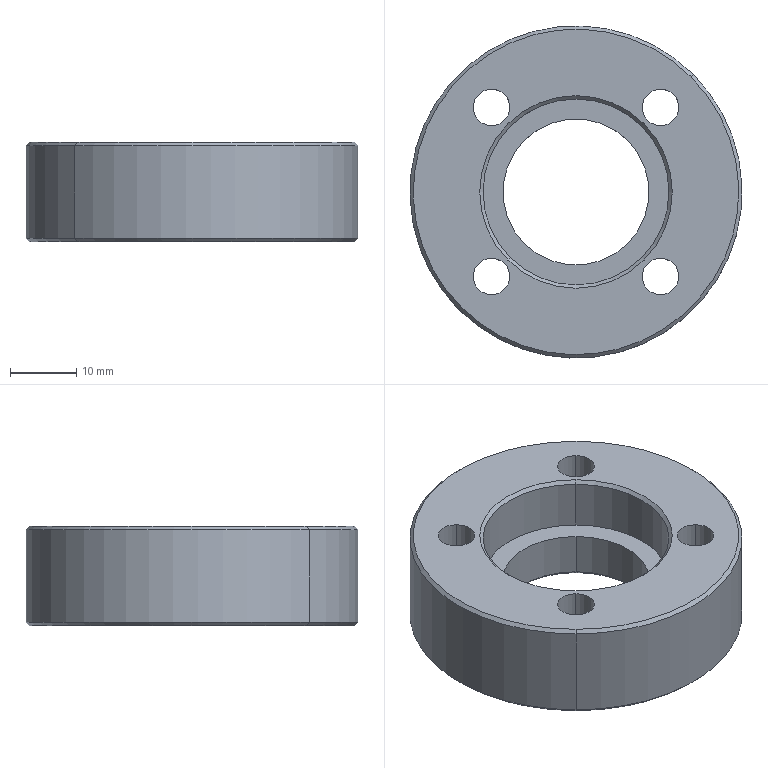Component | SolidWorks | SL010-LeftStreamline-1-1_SL010-2M-0112-000-2-1-1_SL010-LXFB-0102009-1-1 | 1 solid | 37 faces | box 50 x 50 x 15 mm | volume 19198 mm3 | cylinder 22 | cone 8 | plane 7 | commonest cylinder face diameters 10 x8 5.5 x8 22 x2 28 x2 50 x2 | material Aluminum-6061
STEP:
#1=COLOUR_RGB('',0.7922,0.8196,0.9333);
#2=FILL_AREA_STYLE_COLOUR('',#1);
#3=FILL_AREA_STYLE('',(#2));
#4=SURFACE_STYLE_FILL_AREA(#3);
#5=SURFACE_SIDE_STYLE('',(#4));
#6=SURFACE_STYLE_USAGE(.BOTH.,#5);
#7=PRESENTATION_STYLE_ASSIGNMENT((#6));
#8=CARTESIAN_POINT('',(-7.28,-6.882,-25.927));
#9=VERTEX_POINT('',#8);
#10=CARTESIAN_POINT('',(-6.5,-6.103,-25.927));
#11=VERTEX_POINT('',#10);
#12=CARTESIAN_POINT('',(-6.89,-6.492,-25.927));
#13=DIRECTION('',(0.,-0.,1.));
#14=DIRECTION('',(0.7071,0.7071,0.));
#15=AXIS2_PLACEMENT_3D('',#12,#13,#14);
#16=CIRCLE('',#15,0.5512);
#17=EDGE_CURVE('',#9,#11,#16,.T.);
#18=ORIENTED_EDGE('',*,*,#17,.F.);
#19=CARTESIAN_POINT('',(-7.293,-6.896,-25.907));
#20=VERTEX_POINT('',#19);
#21=CARTESIAN_POINT('',(-7.28,-6.882,-25.927));
#22=DIRECTION('',(-0.5,-0.5,0.7071));
#23=VECTOR('',#22,39.37);
#24=LINE('',#21,#23);
#25=EDGE_CURVE('',#9,#20,#24,.T.);
#26=ORIENTED_EDGE('',*,*,#25,.T.);
#27=CARTESIAN_POINT('',(-6.486,-6.089,-25.907));
#28=VERTEX_POINT('',#27);
#29=CARTESIAN_POINT('',(-6.89,-6.492,-25.907));
#30=DIRECTION('',(-0.,0.,-1.));
#31=DIRECTION('',(0.7071,0.7071,0.));
#32=AXIS2_PLACEMENT_3D('',#29,#30,#31);
#33=CIRCLE('',#32,0.5709);
#34=EDGE_CURVE('',#28,#20,#33,.T.);
#35=ORIENTED_EDGE('',*,*,#34,.F.);
#36=CARTESIAN_POINT('',(-6.5,-6.103,-25.927));
#37=DIRECTION('',(0.5,0.5,0.7071));
#38=VECTOR('',#37,39.37);
#39=LINE('',#36,#38);
#40=EDGE_CURVE('',#11,#28,#39,.T.);
#41=ORIENTED_EDGE('',*,*,#40,.F.);
#42=EDGE_LOOP('',(#18,#26,#35,#41));
#43=FACE_OUTER_BOUND('',#42,.T.);
#44=CARTESIAN_POINT('',(-6.89,-6.492,-25.927));
#45=DIRECTION('',(0.,-0.,1.));
#46=DIRECTION('',(0.7071,0.7071,0.));
#47=AXIS2_PLACEMENT_3D('',#44,#45,#46);
#48=CONICAL_SURFACE('',#47,0.5512,0.7854);
#49=ADVANCED_FACE('',(#43),#48,.F.);
#50=CARTESIAN_POINT('',(-6.584,-6.186,-26.478));
#51=VERTEX_POINT('',#50);
#52=CARTESIAN_POINT('',(-7.196,-6.799,-26.478));
#53=VERTEX_POINT('',#52);
#54=CARTESIAN_POINT('',(-6.89,-6.492,-26.478));
#55=DIRECTION('',(-0.,0.,-1.));
#56=DIRECTION('',(0.7071,0.7071,0.));
#57=AXIS2_PLACEMENT_3D('',#54,#55,#56);
#58=CIRCLE('',#57,0.4331);
#59=EDGE_CURVE('',#51,#53,#58,.T.);
#60=ORIENTED_EDGE('',*,*,#59,.F.);
#61=CARTESIAN_POINT('',(-6.57,-6.172,-26.497));
#62=VERTEX_POINT('',#61);
#63=CARTESIAN_POINT('',(-6.57,-6.172,-26.497));
#64=DIRECTION('',(0.5,0.5,-0.7071));
#65=VECTOR('',#64,39.37);
#66=LINE('',#63,#65);
#67=EDGE_CURVE('',#51,#62,#66,.T.);
#68=ORIENTED_EDGE('',*,*,#67,.T.);
#69=CARTESIAN_POINT('',(-7.21,-6.812,-26.497));
#70=VERTEX_POINT('',#69);
#71=CARTESIAN_POINT('',(-6.89,-6.492,-26.497));
#72=DIRECTION('',(0.,-0.,1.));
#73=DIRECTION('',(0.7071,0.7071,0.));
#74=AXIS2_PLACEMENT_3D('',#71,#72,#73);
#75=CIRCLE('',#74,0.4528);
#76=EDGE_CURVE('',#70,#62,#75,.T.);
#77=ORIENTED_EDGE('',*,*,#76,.F.);
#78=CARTESIAN_POINT('',(-7.21,-6.812,-26.497));
#79=DIRECTION('',(-0.5,-0.5,-0.7071));
#80=VECTOR('',#79,39.37);
#81=LINE('',#78,#80);
#82=EDGE_CURVE('',#53,#70,#81,.T.);
#83=ORIENTED_EDGE('',*,*,#82,.F.);
#84=EDGE_LOOP('',(#60,#68,#77,#83));
#85=FACE_OUTER_BOUND('',#84,.T.);
#86=CARTESIAN_POINT('',(-6.89,-6.492,-26.497));
#87=DIRECTION('',(-0.,0.,-1.));
#88=DIRECTION('',(-0.7071,-0.7071,0.));
#89=AXIS2_PLACEMENT_3D('',#86,#87,#88);
#90=CONICAL_SURFACE('',#89,0.4528,0.7854);
#91=ADVANCED_FACE('',(#85),#90,.F.);
#92=CARTESIAN_POINT('',(-6.208,-5.81,-25.907));
#93=VERTEX_POINT('',#92);
#94=CARTESIAN_POINT('',(-7.572,-7.174,-25.907));
#95=VERTEX_POINT('',#94);
#96=CARTESIAN_POINT('',(-6.89,-6.492,-25.907));
#97=DIRECTION('',(0.,-0.,1.));
#98=DIRECTION('',(0.7071,0.7071,0.));
#99=AXIS2_PLACEMENT_3D('',#96,#97,#98);
#100=CIRCLE('',#99,0.9646);
#101=EDGE_CURVE('',#93,#95,#100,.T.);
#102=ORIENTED_EDGE('',*,*,#101,.F.);
#103=CARTESIAN_POINT('',(-6.194,-5.796,-25.927));
#104=VERTEX_POINT('',#103);
#105=CARTESIAN_POINT('',(-6.208,-5.81,-25.907));
#106=DIRECTION('',(0.5,0.5,-0.7071));
#107=VECTOR('',#106,39.37);
#108=LINE('',#105,#107);
#109=EDGE_CURVE('',#93,#104,#108,.T.);
#110=ORIENTED_EDGE('',*,*,#109,.T.);
#111=CARTESIAN_POINT('',(-7.586,-7.188,-25.927));
#112=VERTEX_POINT('',#111);
#113=CARTESIAN_POINT('',(-6.89,-6.492,-25.927));
#114=DIRECTION('',(-0.,0.,-1.));
#115=DIRECTION('',(0.7071,0.7071,0.));
#116=AXIS2_PLACEMENT_3D('',#113,#114,#115);
#117=CIRCLE('',#116,0.9843);
#118=EDGE_CURVE('',#112,#104,#117,.T.);
#119=ORIENTED_EDGE('',*,*,#118,.F.);
#120=CARTESIAN_POINT('',(-7.572,-7.174,-25.907));
#121=DIRECTION('',(-0.5,-0.5,-0.7071));
#122=VECTOR('',#121,39.37);
#123=LINE('',#120,#122);
#124=EDGE_CURVE('',#95,#112,#123,.T.);
#125=ORIENTED_EDGE('',*,*,#124,.F.);
#126=EDGE_LOOP('',(#102,#110,#119,#125));
#127=FACE_OUTER_BOUND('',#126,.T.);
#128=CARTESIAN_POINT('',(-6.89,-6.492,-25.907));
#129=DIRECTION('',(-0.,0.,-1.));
#130=DIRECTION('',(-0.7071,-0.7071,0.));
#131=AXIS2_PLACEMENT_3D('',#128,#129,#130);
#132=CONICAL_SURFACE('',#131,0.9646,0.7854);
#133=ADVANCED_FACE('',(#127),#132,.T.);
#134=CARTESIAN_POINT('',(-7.572,-7.174,-26.497));
#135=VERTEX_POINT('',#134);
#136=CARTESIAN_POINT('',(-6.208,-5.81,-26.497));
#137=VERTEX_POINT('',#136);
#138=CARTESIAN_POINT('',(-6.89,-6.492,-26.497));
#139=DIRECTION('',(-0.,0.,-1.));
#140=DIRECTION('',(0.7071,0.7071,0.));
#141=AXIS2_PLACEMENT_3D('',#138,#139,#140);
#142=CIRCLE('',#141,0.9646);
#143=EDGE_CURVE('',#135,#137,#142,.T.);
#144=ORIENTED_EDGE('',*,*,#143,.F.);
#145=CARTESIAN_POINT('',(-7.586,-7.188,-26.478));
#146=VERTEX_POINT('',#145);
#147=CARTESIAN_POINT('',(-7.586,-7.188,-26.478));
#148=DIRECTION('',(-0.5,-0.5,0.7071));
#149=VECTOR('',#148,39.37);
#150=LINE('',#147,#149);
#151=EDGE_CURVE('',#135,#146,#150,.T.);
#152=ORIENTED_EDGE('',*,*,#151,.T.);
#153=CARTESIAN_POINT('',(-6.194,-5.796,-26.478));
#154=VERTEX_POINT('',#153);
#155=CARTESIAN_POINT('',(-6.89,-6.492,-26.478));
#156=DIRECTION('',(0.,-0.,1.));
#157=DIRECTION('',(0.7071,0.7071,0.));
#158=AXIS2_PLACEMENT_3D('',#155,#156,#157);
#159=CIRCLE('',#158,0.9843);
#160=EDGE_CURVE('',#154,#146,#159,.T.);
#161=ORIENTED_EDGE('',*,*,#160,.F.);
#162=CARTESIAN_POINT('',(-6.194,-5.796,-26.478));
#163=DIRECTION('',(0.5,0.5,0.7071));
#164=VECTOR('',#163,39.37);
#165=LINE('',#162,#164);
#166=EDGE_CURVE('',#137,#154,#165,.T.);
#167=ORIENTED_EDGE('',*,*,#166,.F.);
#168=EDGE_LOOP('',(#144,#152,#161,#167));
#169=FACE_OUTER_BOUND('',#168,.T.);
#170=CARTESIAN_POINT('',(-6.89,-6.492,-26.478));
#171=DIRECTION('',(0.,-0.,1.));
#172=DIRECTION('',(0.7071,0.7071,0.));
#173=AXIS2_PLACEMENT_3D('',#170,#171,#172);
#174=CONICAL_SURFACE('',#173,0.9843,0.7854);
#175=ADVANCED_FACE('',(#169),#174,.T.);
#176=CARTESIAN_POINT('',(-7.252,-5.852,-26.285));
#177=VERTEX_POINT('',#176);
#178=CARTESIAN_POINT('',(-7.53,-6.13,-26.285));
#179=VERTEX_POINT('',#178);
#180=CARTESIAN_POINT('',(-7.391,-5.991,-26.285));
#181=DIRECTION('',(-0.,0.,-1.));
#182=DIRECTION('',(-0.7071,-0.7071,0.));
#183=AXIS2_PLACEMENT_3D('',#180,#181,#182);
#184=CIRCLE('',#183,0.1969);
#185=EDGE_CURVE('',#177,#179,#184,.T.);
#186=ORIENTED_EDGE('',*,*,#185,.F.);
#187=CARTESIAN_POINT('',(-7.252,-5.852,-26.497));
#188=VERTEX_POINT('',#187);
#189=CARTESIAN_POINT('',(-7.252,-5.852,-26.497));
#190=DIRECTION('',(-0.,0.,-1.));
#191=VECTOR('',#190,39.37);
#192=LINE('',#189,#191);
#193=EDGE_CURVE('',#177,#188,#192,.T.);
#194=ORIENTED_EDGE('',*,*,#193,.T.);
#195=CARTESIAN_POINT('',(-7.53,-6.13,-26.497));
#196=VERTEX_POINT('',#195);
#197=CARTESIAN_POINT('',(-7.391,-5.991,-26.497));
#198=DIRECTION('',(-0.,0.,-1.));
#199=DIRECTION('',(-0.7071,-0.7071,0.));
#200=AXIS2_PLACEMENT_3D('',#197,#198,#199);
#201=CIRCLE('',#200,0.1969);
#202=EDGE_CURVE('',#188,#196,#201,.T.);
#203=ORIENTED_EDGE('',*,*,#202,.T.);
#204=CARTESIAN_POINT('',(-7.53,-6.13,-26.497));
#205=DIRECTION('',(-0.,0.,-1.));
#206=VECTOR('',#205,39.37);
#207=LINE('',#204,#206);
#208=EDGE_CURVE('',#179,#196,#207,.T.);
#209=ORIENTED_EDGE('',*,*,#208,.F.);
#210=EDGE_LOOP('',(#186,#194,#203,#209));
#211=FACE_OUTER_BOUND('',#210,.T.);
#212=CARTESIAN_POINT('',(-7.391,-5.991,-26.497));
#213=DIRECTION('',(-0.,0.,-1.));
#214=DIRECTION('',(-0.7071,-0.7071,0.));
#215=AXIS2_PLACEMENT_3D('',#212,#213,#214);
#216=CYLINDRICAL_SURFACE('',#215,0.1969);
#217=ADVANCED_FACE('',(#211),#216,.F.);
#218=CARTESIAN_POINT('',(-7.314,-5.915,-25.907));
#219=VERTEX_POINT('',#218);
#220=CARTESIAN_POINT('',(-7.467,-6.068,-25.907));
#221=VERTEX_POINT('',#220);
#222=CARTESIAN_POINT('',(-7.391,-5.991,-25.907));
#223=DIRECTION('',(-0.,0.,-1.));
#224=DIRECTION('',(-0.7071,-0.7071,0.));
#225=AXIS2_PLACEMENT_3D('',#222,#223,#224);
#226=CIRCLE('',#225,0.1083);
#227=EDGE_CURVE('',#219,#221,#226,.T.);
#228=ORIENTED_EDGE('',*,*,#227,.F.);
#229=CARTESIAN_POINT('',(-7.314,-5.915,-26.285));
#230=VERTEX_POINT('',#229);
#231=CARTESIAN_POINT('',(-7.314,-5.915,-26.497));
#232=DIRECTION('',(-0.,0.,-1.));
#233=VECTOR('',#232,39.37);
#234=LINE('',#231,#233);
#235=EDGE_CURVE('',#219,#230,#234,.T.);
#236=ORIENTED_EDGE('',*,*,#235,.T.);
#237=CARTESIAN_POINT('',(-7.467,-6.068,-26.285));
#238=VERTEX_POINT('',#237);
#239=CARTESIAN_POINT('',(-7.391,-5.991,-26.285));
#240=DIRECTION('',(-0.,0.,-1.));
#241=DIRECTION('',(-0.7071,-0.7071,0.));
#242=AXIS2_PLACEMENT_3D('',#239,#240,#241);
#243=CIRCLE('',#242,0.1083);
#244=EDGE_CURVE('',#230,#238,#243,.T.);
#245=ORIENTED_EDGE('',*,*,#244,.T.);
#246=CARTESIAN_POINT('',(-7.467,-6.068,-26.497));
#247=DIRECTION('',(-0.,0.,-1.));
#248=VECTOR('',#247,39.37);
#249=LINE('',#246,#248);
#250=EDGE_CURVE('',#221,#238,#249,.T.);
#251=ORIENTED_EDGE('',*,*,#250,.F.);
#252=EDGE_LOOP('',(#228,#236,#245,#251));
#253=FACE_OUTER_BOUND('',#252,.T.);
#254=CARTESIAN_POINT('',(-7.391,-5.991,-26.497));
#255=DIRECTION('',(-0.,0.,-1.));
#256=DIRECTION('',(-0.7071,-0.7071,0.));
#257=AXIS2_PLACEMENT_3D('',#254,#255,#256);
#258=CYLINDRICAL_SURFACE('',#257,0.1083);
#259=ADVANCED_FACE('',(#253),#258,.F.);
#260=CARTESIAN_POINT('',(-6.249,-5.852,-26.285));
#261=VERTEX_POINT('',#260);
#262=CARTESIAN_POINT('',(-6.528,-6.13,-26.285));
#263=VERTEX_POINT('',#262);
#264=CARTESIAN_POINT('',(-6.389,-5.991,-26.285));
#265=DIRECTION('',(-0.,0.,-1.));
#266=DIRECTION('',(-0.7071,-0.7071,0.));
#267=AXIS2_PLACEMENT_3D('',#264,#265,#266);
#268=CIRCLE('',#267,0.1969);
#269=EDGE_CURVE('',#261,#263,#268,.T.);
#270=ORIENTED_EDGE('',*,*,#269,.F.);
#271=CARTESIAN_POINT('',(-6.249,-5.852,-26.497));
#272=VERTEX_POINT('',#271);
#273=CARTESIAN_POINT('',(-6.249,-5.852,-26.497));
#274=DIRECTION('',(-0.,0.,-1.));
#275=VECTOR('',#274,39.37);
#276=LINE('',#273,#275);
#277=EDGE_CURVE('',#261,#272,#276,.T.);
#278=ORIENTED_EDGE('',*,*,#277,.T.);
#279=CARTESIAN_POINT('',(-6.528,-6.13,-26.497));
#280=VERTEX_POINT('',#279);
#281=CARTESIAN_POINT('',(-6.389,-5.991,-26.497));
#282=DIRECTION('',(-0.,0.,-1.));
#283=DIRECTION('',(-0.7071,-0.7071,0.));
#284=AXIS2_PLACEMENT_3D('',#281,#282,#283);
#285=CIRCLE('',#284,0.1969);
#286=EDGE_CURVE('',#272,#280,#285,.T.);
#287=ORIENTED_EDGE('',*,*,#286,.T.);
#288=CARTESIAN_POINT('',(-6.528,-6.13,-26.497));
#289=DIRECTION('',(-0.,0.,-1.));
#290=VECTOR('',#289,39.37);
#291=LINE('',#288,#290);
#292=EDGE_CURVE('',#263,#280,#291,.T.);
#293=ORIENTED_EDGE('',*,*,#292,.F.);
#294=EDGE_LOOP('',(#270,#278,#287,#293));
#295=FACE_OUTER_BOUND('',#294,.T.);
#296=CARTESIAN_POINT('',(-6.389,-5.991,-26.497));
#297=DIRECTION('',(-0.,0.,-1.));
#298=DIRECTION('',(-0.7071,-0.7071,0.));
#299=AXIS2_PLACEMENT_3D('',#296,#297,#298);
#300=CYLINDRICAL_SURFACE('',#299,0.1969);
#301=ADVANCED_FACE('',(#295),#300,.F.);
#302=CARTESIAN_POINT('',(-6.312,-5.915,-25.907));
#303=VERTEX_POINT('',#302);
#304=CARTESIAN_POINT('',(-6.465,-6.068,-25.907));
#305=VERTEX_POINT('',#304);
#306=CARTESIAN_POINT('',(-6.389,-5.991,-25.907));
#307=DIRECTION('',(-0.,0.,-1.));
#308=DIRECTION('',(-0.7071,-0.7071,0.));
#309=AXIS2_PLACEMENT_3D('',#306,#307,#308);
#310=CIRCLE('',#309,0.1083);
#311=EDGE_CURVE('',#303,#305,#310,.T.);
#312=ORIENTED_EDGE('',*,*,#311,.F.);
#313=CARTESIAN_POINT('',(-6.312,-5.915,-26.285));
#314=VERTEX_POINT('',#313);
#315=CARTESIAN_POINT('',(-6.312,-5.915,-26.497));
#316=DIRECTION('',(-0.,0.,-1.));
#317=VECTOR('',#316,39.37);
#318=LINE('',#315,#317);
#319=EDGE_CURVE('',#303,#314,#318,.T.);
#320=ORIENTED_EDGE('',*,*,#319,.T.);
#321=CARTESIAN_POINT('',(-6.465,-6.068,-26.285));
#322=VERTEX_POINT('',#321);
#323=CARTESIAN_POINT('',(-6.389,-5.991,-26.285));
#324=DIRECTION('',(-0.,0.,-1.));
#325=DIRECTION('',(-0.7071,-0.7071,0.));
#326=AXIS2_PLACEMENT_3D('',#323,#324,#325);
#327=CIRCLE('',#326,0.1083);
#328=EDGE_CURVE('',#314,#322,#327,.T.);
#329=ORIENTED_EDGE('',*,*,#328,.T.);
#330=CARTESIAN_POINT('',(-6.465,-6.068,-26.497));
#331=DIRECTION('',(-0.,0.,-1.));
#332=VECTOR('',#331,39.37);
#333=LINE('',#330,#332);
#334=EDGE_CURVE('',#305,#322,#333,.T.);
#335=ORIENTED_EDGE('',*,*,#334,.F.);
#336=EDGE_LOOP('',(#312,#320,#329,#335));
#337=FACE_OUTER_BOUND('',#336,.T.);
#338=CARTESIAN_POINT('',(-6.389,-5.991,-26.497));
#339=DIRECTION('',(-0.,0.,-1.));
#340=DIRECTION('',(-0.7071,-0.7071,0.));
#341=AXIS2_PLACEMENT_3D('',#338,#339,#340);
#342=CYLINDRICAL_SURFACE('',#341,0.1083);
#343=ADVANCED_FACE('',(#337),#342,.F.);
#344=CARTESIAN_POINT('',(-6.249,-6.854,-26.285));
#345=VERTEX_POINT('',#344);
#346=CARTESIAN_POINT('',(-6.528,-7.133,-26.285));
#347=VERTEX_POINT('',#346);
#348=CARTESIAN_POINT('',(-6.389,-6.993,-26.285));
#349=DIRECTION('',(-0.,0.,-1.));
#350=DIRECTION('',(-0.7071,-0.7071,0.));
#351=AXIS2_PLACEMENT_3D('',#348,#349,#350);
#352=CIRCLE('',#351,0.1969);
#353=EDGE_CURVE('',#345,#347,#352,.T.);
#354=ORIENTED_EDGE('',*,*,#353,.F.);
#355=CARTESIAN_POINT('',(-6.249,-6.854,-26.497));
#356=VERTEX_POINT('',#355);
#357=CARTESIAN_POINT('',(-6.249,-6.854,-26.497));
#358=DIRECTION('',(-0.,0.,-1.));
#359=VECTOR('',#358,39.37);
#360=LINE('',#357,#359);
#361=EDGE_CURVE('',#345,#356,#360,.T.);
#362=ORIENTED_EDGE('',*,*,#361,.T.);
#363=CARTESIAN_POINT('',(-6.528,-7.133,-26.497));
#364=VERTEX_POINT('',#363);
#365=CARTESIAN_POINT('',(-6.389,-6.993,-26.497));
#366=DIRECTION('',(-0.,0.,-1.));
#367=DIRECTION('',(-0.7071,-0.7071,0.));
#368=AXIS2_PLACEMENT_3D('',#365,#366,#367);
#369=CIRCLE('',#368,0.1969);
#370=EDGE_CURVE('',#356,#364,#369,.T.);
#371=ORIENTED_EDGE('',*,*,#370,.T.);
#372=CARTESIAN_POINT('',(-6.528,-7.133,-26.497));
#373=DIRECTION('',(-0.,0.,-1.));
#374=VECTOR('',#373,39.37);
#375=LINE('',#372,#374);
#376=EDGE_CURVE('',#347,#364,#375,.T.);
#377=ORIENTED_EDGE('',*,*,#376,.F.);
#378=EDGE_LOOP('',(#354,#362,#371,#377));
#379=FACE_OUTER_BOUND('',#378,.T.);
#380=CARTESIAN_POINT('',(-6.389,-6.993,-26.497));
#381=DIRECTION('',(-0.,0.,-1.));
#382=DIRECTION('',(-0.7071,-0.7071,0.));
#383=AXIS2_PLACEMENT_3D('',#380,#381,#382);
#384=CYLINDRICAL_SURFACE('',#383,0.1969);
#385=ADVANCED_FACE('',(#379),#384,.F.);
#386=CARTESIAN_POINT('',(-6.312,-6.917,-25.907));
#387=VERTEX_POINT('',#386);
#388=CARTESIAN_POINT('',(-6.465,-7.07,-25.907));
#389=VERTEX_POINT('',#388);
#390=CARTESIAN_POINT('',(-6.389,-6.993,-25.907));
#391=DIRECTION('',(-0.,0.,-1.));
#392=DIRECTION('',(-0.7071,-0.7071,0.));
#393=AXIS2_PLACEMENT_3D('',#390,#391,#392);
#394=CIRCLE('',#393,0.1083);
#395=EDGE_CURVE('',#387,#389,#394,.T.);
#396=ORIENTED_EDGE('',*,*,#395,.F.);
#397=CARTESIAN_POINT('',(-6.312,-6.917,-26.285));
#398=VERTEX_POINT('',#397);
#399=CARTESIAN_POINT('',(-6.312,-6.917,-26.497));
#400=DIRECTION('',(-0.,0.,-1.));
#401=VECTOR('',#400,39.37);
#402=LINE('',#399,#401);
#403=EDGE_CURVE('',#387,#398,#402,.T.);
#404=ORIENTED_EDGE('',*,*,#403,.T.);
#405=CARTESIAN_POINT('',(-6.465,-7.07,-26.285));
#406=VERTEX_POINT('',#405);
#407=CARTESIAN_POINT('',(-6.389,-6.993,-26.285));
#408=DIRECTION('',(-0.,0.,-1.));
#409=DIRECTION('',(-0.7071,-0.7071,0.));
#410=AXIS2_PLACEMENT_3D('',#407,#408,#409);
#411=CIRCLE('',#410,0.1083);
#412=EDGE_CURVE('',#398,#406,#411,.T.);
#413=ORIENTED_EDGE('',*,*,#412,.T.);
#414=CARTESIAN_POINT('',(-6.465,-7.07,-26.497));
#415=DIRECTION('',(-0.,0.,-1.));
#416=VECTOR('',#415,39.37);
#417=LINE('',#414,#416);
#418=EDGE_CURVE('',#389,#406,#417,.T.);
#419=ORIENTED_EDGE('',*,*,#418,.F.);
#420=EDGE_LOOP('',(#396,#404,#413,#419));
#421=FACE_OUTER_BOUND('',#420,.T.);
#422=CARTESIAN_POINT('',(-6.389,-6.993,-26.497));
#423=DIRECTION('',(-0.,0.,-1.));
#424=DIRECTION('',(-0.7071,-0.7071,0.));
#425=AXIS2_PLACEMENT_3D('',#422,#423,#424);
#426=CYLINDRICAL_SURFACE('',#425,0.1083);
#427=ADVANCED_FACE('',(#421),#426,.F.);
#428=CARTESIAN_POINT('',(-7.252,-6.854,-26.285));
#429=VERTEX_POINT('',#428);
#430=CARTESIAN_POINT('',(-7.53,-7.133,-26.285));
#431=VERTEX_POINT('',#430);
#432=CARTESIAN_POINT('',(-7.391,-6.993,-26.285));
#433=DIRECTION('',(-0.,0.,-1.));
#434=DIRECTION('',(-0.7071,-0.7071,0.));
#435=AXIS2_PLACEMENT_3D('',#432,#433,#434);
#436=CIRCLE('',#435,0.1969);
#437=EDGE_CURVE('',#429,#431,#436,.T.);
#438=ORIENTED_EDGE('',*,*,#437,.F.);
#439=CARTESIAN_POINT('',(-7.252,-6.854,-26.497));
#440=VERTEX_POINT('',#439);
#441=CARTESIAN_POINT('',(-7.252,-6.854,-26.497));
#442=DIRECTION('',(-0.,0.,-1.));
#443=VECTOR('',#442,39.37);
#444=LINE('',#441,#443);
#445=EDGE_CURVE('',#429,#440,#444,.T.);
#446=ORIENTED_EDGE('',*,*,#445,.T.);
#447=CARTESIAN_POINT('',(-7.53,-7.133,-26.497));
#448=VERTEX_POINT('',#447);
#449=CARTESIAN_POINT('',(-7.391,-6.993,-26.497));
#450=DIRECTION('',(-0.,0.,-1.));
#451=DIRECTION('',(-0.7071,-0.7071,0.));
#452=AXIS2_PLACEMENT_3D('',#449,#450,#451);
#453=CIRCLE('',#452,0.1969);
#454=EDGE_CURVE('',#440,#448,#453,.T.);
#455=ORIENTED_EDGE('',*,*,#454,.T.);
#456=CARTESIAN_POINT('',(-7.53,-7.133,-26.497));
#457=DIRECTION('',(-0.,0.,-1.));
#458=VECTOR('',#457,39.37);
#459=LINE('',#456,#458);
#460=EDGE_CURVE('',#431,#448,#459,.T.);
#461=ORIENTED_EDGE('',*,*,#460,.F.);
#462=EDGE_LOOP('',(#438,#446,#455,#461));
#463=FACE_OUTER_BOUND('',#462,.T.);
#464=CARTESIAN_POINT('',(-7.391,-6.993,-26.497));
#465=DIRECTION('',(-0.,0.,-1.));
#466=DIRECTION('',(-0.7071,-0.7071,0.));
#467=AXIS2_PLACEMENT_3D('',#464,#465,#466);
#468=CYLINDRICAL_SURFACE('',#467,0.1969);
#469=ADVANCED_FACE('',(#463),#468,.F.);
#470=CARTESIAN_POINT('',(-7.314,-6.917,-25.907));
#471=VERTEX_POINT('',#470);
#472=CARTESIAN_POINT('',(-7.467,-7.07,-25.907));
#473=VERTEX_POINT('',#472);
#474=CARTESIAN_POINT('',(-7.391,-6.993,-25.907));
#475=DIRECTION('',(-0.,0.,-1.));
#476=DIRECTION('',(-0.7071,-0.7071,0.));
#477=AXIS2_PLACEMENT_3D('',#474,#475,#476);
#478=CIRCLE('',#477,0.1083);
#479=EDGE_CURVE('',#471,#473,#478,.T.);
#480=ORIENTED_EDGE('',*,*,#479,.F.);
#481=CARTESIAN_POINT('',(-7.314,-6.917,-26.285));
#482=VERTEX_POINT('',#481);
#483=CARTESIAN_POINT('',(-7.314,-6.917,-26.497));
#484=DIRECTION('',(-0.,0.,-1.));
#485=VECTOR('',#484,39.37);
#486=LINE('',#483,#485);
#487=EDGE_CURVE('',#471,#482,#486,.T.);
#488=ORIENTED_EDGE('',*,*,#487,.T.);
#489=CARTESIAN_POINT('',(-7.467,-7.07,-26.285));
#490=VERTEX_POINT('',#489);
#491=CARTESIAN_POINT('',(-7.391,-6.993,-26.285));
#492=DIRECTION('',(-0.,0.,-1.));
#493=DIRECTION('',(-0.7071,-0.7071,0.));
#494=AXIS2_PLACEMENT_3D('',#491,#492,#493);
#495=CIRCLE('',#494,0.1083);
#496=EDGE_CURVE('',#482,#490,#495,.T.);
#497=ORIENTED_EDGE('',*,*,#496,.T.);
#498=CARTESIAN_POINT('',(-7.467,-7.07,-26.497));
#499=DIRECTION('',(-0.,0.,-1.));
#500=VECTOR('',#499,39.37);
#501=LINE('',#498,#500);
#502=EDGE_CURVE('',#473,#490,#501,.T.);
#503=ORIENTED_EDGE('',*,*,#502,.F.);
#504=EDGE_LOOP('',(#480,#488,#497,#503));
#505=FACE_OUTER_BOUND('',#504,.T.);
#506=CARTESIAN_POINT('',(-7.391,-6.993,-26.497));
#507=DIRECTION('',(-0.,0.,-1.));
#508=DIRECTION('',(-0.7071,-0.7071,0.));
#509=AXIS2_PLACEMENT_3D('',#506,#507,#508);
#510=CYLINDRICAL_SURFACE('',#509,0.1083);
#511=ADVANCED_FACE('',(#505),#510,.F.);
#512=ORIENTED_EDGE('',*,*,#59,.T.);
#513=CARTESIAN_POINT('',(-7.196,-6.799,-26.222));
#514=VERTEX_POINT('',#513);
#515=CARTESIAN_POINT('',(-7.196,-6.799,-26.497));
#516=DIRECTION('',(0.,-0.,1.));
#517=VECTOR('',#516,39.37);
#518=LINE('',#515,#517);
#519=EDGE_CURVE('',#53,#514,#518,.T.);
#520=ORIENTED_EDGE('',*,*,#519,.T.);
#521=CARTESIAN_POINT('',(-6.584,-6.186,-26.222));
#522=VERTEX_POINT('',#521);
#523=CARTESIAN_POINT('',(-6.89,-6.492,-26.222));
#524=DIRECTION('',(0.,-0.,1.));
#525=DIRECTION('',(0.7071,0.7071,0.));
#526=AXIS2_PLACEMENT_3D('',#523,#524,#525);
#527=CIRCLE('',#526,0.4331);
#528=EDGE_CURVE('',#514,#522,#527,.T.);
#529=ORIENTED_EDGE('',*,*,#528,.T.);
#530=CARTESIAN_POINT('',(-6.584,-6.186,-26.497));
#531=DIRECTION('',(0.,-0.,1.));
#532=VECTOR('',#531,39.37);
#533=LINE('',#530,#532);
#534=EDGE_CURVE('',#51,#522,#533,.T.);
#535=ORIENTED_EDGE('',*,*,#534,.F.);
#536=EDGE_LOOP('',(#512,#520,#529,#535));
#537=FACE_OUTER_BOUND('',#536,.T.);
#538=CARTESIAN_POINT('',(-6.89,-6.492,-26.497));
#539=DIRECTION('',(0.,-0.,1.));
#540=DIRECTION('',(0.7071,0.7071,0.));
#541=AXIS2_PLACEMENT_3D('',#538,#539,#540);
#542=CYLINDRICAL_SURFACE('',#541,0.4331);
#543=ADVANCED_FACE('',(#537),#542,.F.);
#544=CARTESIAN_POINT('',(-7.28,-6.882,-26.222));
#545=VERTEX_POINT('',#544);
#546=CARTESIAN_POINT('',(-6.5,-6.103,-26.222));
#547=VERTEX_POINT('',#546);
#548=CARTESIAN_POINT('',(-6.89,-6.492,-26.222));
#549=DIRECTION('',(0.,-0.,1.));
#550=DIRECTION('',(0.7071,0.7071,0.));
#551=AXIS2_PLACEMENT_3D('',#548,#549,#550);
#552=CIRCLE('',#551,0.5512);
#553=EDGE_CURVE('',#545,#547,#552,.T.);
#554=ORIENTED_EDGE('',*,*,#553,.F.);
#555=CARTESIAN_POINT('',(-7.28,-6.882,-26.222));
#556=DIRECTION('',(0.,-0.,1.));
#557=VECTOR('',#556,39.37);
#558=LINE('',#555,#557);
#559=EDGE_CURVE('',#545,#9,#558,.T.);
#560=ORIENTED_EDGE('',*,*,#559,.T.);
#561=ORIENTED_EDGE('',*,*,#17,.T.);
#562=CARTESIAN_POINT('',(-6.5,-6.103,-26.222));
#563=DIRECTION('',(0.,-0.,1.));
#564=VECTOR('',#563,39.37);
#565=LINE('',#562,#564);
#566=EDGE_CURVE('',#547,#11,#565,.T.);
#567=ORIENTED_EDGE('',*,*,#566,.F.);
#568=EDGE_LOOP('',(#554,#560,#561,#567));
#569=FACE_OUTER_BOUND('',#568,.T.);
#570=CARTESIAN_POINT('',(-6.89,-6.492,-26.222));
#571=DIRECTION('',(0.,-0.,1.));
#572=DIRECTION('',(0.7071,0.7071,0.));
#573=AXIS2_PLACEMENT_3D('',#570,#571,#572);
#574=CYLINDRICAL_SURFACE('',#573,0.5512);
#575=ADVANCED_FACE('',(#569),#574,.F.);
#576=ORIENTED_EDGE('',*,*,#118,.T.);
#577=CARTESIAN_POINT('',(-6.194,-5.796,-25.907));
#578=DIRECTION('',(-0.,0.,-1.));
#579=VECTOR('',#578,39.37);
#580=LINE('',#577,#579);
#581=EDGE_CURVE('',#104,#154,#580,.T.);
#582=ORIENTED_EDGE('',*,*,#581,.T.);
#583=ORIENTED_EDGE('',*,*,#160,.T.);
#584=CARTESIAN_POINT('',(-7.586,-7.188,-25.907));
#585=DIRECTION('',(-0.,0.,-1.));
#586=VECTOR('',#585,39.37);
#587=LINE('',#584,#586);
#588=EDGE_CURVE('',#112,#146,#587,.T.);
#589=ORIENTED_EDGE('',*,*,#588,.F.);
#590=EDGE_LOOP('',(#576,#582,#583,#589));
#591=FACE_OUTER_BOUND('',#590,.T.);
#592=CARTESIAN_POINT('',(-6.89,-6.492,-25.907));
#593=DIRECTION('',(-0.,0.,-1.));
#594=DIRECTION('',(-0.7071,-0.7071,0.));
#595=AXIS2_PLACEMENT_3D('',#592,#593,#594);
#596=CYLINDRICAL_SURFACE('',#595,0.9843);
#597=ADVANCED_FACE('',(#591),#596,.T.);
#598=ORIENTED_EDGE('',*,*,#581,.F.);
#599=CARTESIAN_POINT('',(-6.89,-6.492,-25.927));
#600=DIRECTION('',(-0.,0.,-1.));
#601=DIRECTION('',(0.7071,0.7071,0.));
#602=AXIS2_PLACEMENT_3D('',#599,#600,#601);
#603=CIRCLE('',#602,0.9843);
#604=EDGE_CURVE('',#104,#112,#603,.T.);
#605=ORIENTED_EDGE('',*,*,#604,.T.);
#606=ORIENTED_EDGE('',*,*,#588,.T.);
#607=CARTESIAN_POINT('',(-6.89,-6.492,-26.478));
#608=DIRECTION('',(0.,-0.,1.));
#609=DIRECTION('',(0.7071,0.7071,0.));
#610=AXIS2_PLACEMENT_3D('',#607,#608,#609);
#611=CIRCLE('',#610,0.9843);
#612=EDGE_CURVE('',#146,#154,#611,.T.);
#613=ORIENTED_EDGE('',*,*,#612,.T.);
#614=EDGE_LOOP('',(#598,#605,#606,#613));
#615=FACE_OUTER_BOUND('',#614,.T.);
#616=CARTESIAN_POINT('',(-6.89,-6.492,-25.907));
#617=DIRECTION('',(-0.,0.,-1.));
#618=DIRECTION('',(-0.7071,-0.7071,0.));
#619=AXIS2_PLACEMENT_3D('',#616,#617,#618);
#620=CYLINDRICAL_SURFACE('',#619,0.9843);
#621=ADVANCED_FACE('',(#615),#620,.T.);
#622=CARTESIAN_POINT('',(-6.89,-6.492,-25.907));
#623=DIRECTION('',(0.,-0.,1.));
#624=DIRECTION('',(0.7071,0.7071,0.));
#625=AXIS2_PLACEMENT_3D('',#622,#623,#624);
#626=CIRCLE('',#625,0.9646);
#627=EDGE_CURVE('',#95,#93,#626,.T.);
#628=ORIENTED_EDGE('',*,*,#627,.T.);
#629=ORIENTED_EDGE('',*,*,#101,.T.);
#630=EDGE_LOOP('',(#628,#629));
#631=FACE_OUTER_BOUND('',#630,.T.);
#632=ORIENTED_EDGE('',*,*,#34,.T.);
#633=CARTESIAN_POINT('',(-6.89,-6.492,-25.907));
#634=DIRECTION('',(-0.,0.,-1.));
#635=DIRECTION('',(0.7071,0.7071,0.));
#636=AXIS2_PLACEMENT_3D('',#633,#634,#635);
#637=CIRCLE('',#636,0.5709);
#638=EDGE_CURVE('',#20,#28,#637,.T.);
#639=ORIENTED_EDGE('',*,*,#638,.T.);
#640=EDGE_LOOP('',(#632,#639));
#641=FACE_BOUND('',#640,.T.);
#642=CARTESIAN_POINT('',(-7.391,-5.991,-25.907));
#643=DIRECTION('',(-0.,0.,-1.));
#644=DIRECTION('',(-0.7071,-0.7071,0.));
#645=AXIS2_PLACEMENT_3D('',#642,#643,#644);
#646=CIRCLE('',#645,0.1083);
#647=EDGE_CURVE('',#221,#219,#646,.T.);
#648=ORIENTED_EDGE('',*,*,#647,.T.);
#649=ORIENTED_EDGE('',*,*,#227,.T.);
#650=EDGE_LOOP('',(#648,#649));
#651=FACE_BOUND('',#650,.T.);
#652=CARTESIAN_POINT('',(-6.389,-5.991,-25.907));
#653=DIRECTION('',(-0.,0.,-1.));
#654=DIRECTION('',(-0.7071,-0.7071,0.));
#655=AXIS2_PLACEMENT_3D('',#652,#653,#654);
#656=CIRCLE('',#655,0.1083);
#657=EDGE_CURVE('',#305,#303,#656,.T.);
#658=ORIENTED_EDGE('',*,*,#657,.T.);
#659=ORIENTED_EDGE('',*,*,#311,.T.);
#660=EDGE_LOOP('',(#658,#659));
#661=FACE_BOUND('',#660,.T.);
#662=CARTESIAN_POINT('',(-6.389,-6.993,-25.907));
#663=DIRECTION('',(-0.,0.,-1.));
#664=DIRECTION('',(-0.7071,-0.7071,0.));
#665=AXIS2_PLACEMENT_3D('',#662,#663,#664);
#666=CIRCLE('',#665,0.1083);
#667=EDGE_CURVE('',#389,#387,#666,.T.);
#668=ORIENTED_EDGE('',*,*,#667,.T.);
#669=ORIENTED_EDGE('',*,*,#395,.T.);
#670=EDGE_LOOP('',(#668,#669));
#671=FACE_BOUND('',#670,.T.);
#672=CARTESIAN_POINT('',(-7.391,-6.993,-25.907));
#673=DIRECTION('',(-0.,0.,-1.));
#674=DIRECTION('',(-0.7071,-0.7071,0.));
#675=AXIS2_PLACEMENT_3D('',#672,#673,#674);
#676=CIRCLE('',#675,0.1083);
#677=EDGE_CURVE('',#473,#471,#676,.T.);
#678=ORIENTED_EDGE('',*,*,#677,.T.);
#679=ORIENTED_EDGE('',*,*,#479,.T.);
#680=EDGE_LOOP('',(#678,#679));
#681=FACE_BOUND('',#680,.T.);
#682=CARTESIAN_POINT('',(-6.89,-6.492,-25.907));
#683=DIRECTION('',(0.,-0.,1.));
#684=DIRECTION('',(0.7071,0.7071,-0.));
#685=AXIS2_PLACEMENT_3D('',#682,#683,#684);
#686=PLANE('',#685);
#687=ADVANCED_FACE('',(#631,#641,#651,#661,#671,#681),#686,.T.);
#688=CARTESIAN_POINT('',(-6.89,-6.492,-26.497));
#689=DIRECTION('',(-0.,0.,-1.));
#690=DIRECTION('',(0.7071,0.7071,0.));
#691=AXIS2_PLACEMENT_3D('',#688,#689,#690);
#692=CIRCLE('',#691,0.9646);
#693=EDGE_CURVE('',#137,#135,#692,.T.);
#694=ORIENTED_EDGE('',*,*,#693,.T.);
#695=ORIENTED_EDGE('',*,*,#143,.T.);
#696=EDGE_LOOP('',(#694,#695));
#697=FACE_OUTER_BOUND('',#696,.T.);
#698=ORIENTED_EDGE('',*,*,#76,.T.);
#699=CARTESIAN_POINT('',(-6.89,-6.492,-26.497));
#700=DIRECTION('',(0.,-0.,1.));
#701=DIRECTION('',(0.7071,0.7071,0.));
#702=AXIS2_PLACEMENT_3D('',#699,#700,#701);
#703=CIRCLE('',#702,0.4528);
#704=EDGE_CURVE('',#62,#70,#703,.T.);
#705=ORIENTED_EDGE('',*,*,#704,.T.);
#706=EDGE_LOOP('',(#698,#705));
#707=FACE_BOUND('',#706,.T.);
#708=CARTESIAN_POINT('',(-7.391,-5.991,-26.497));
#709=DIRECTION('',(-0.,0.,-1.));
#710=DIRECTION('',(-0.7071,-0.7071,0.));
#711=AXIS2_PLACEMENT_3D('',#708,#709,#710);
#712=CIRCLE('',#711,0.1969);
#713=EDGE_CURVE('',#196,#188,#712,.T.);
#714=ORIENTED_EDGE('',*,*,#713,.F.);
#715=ORIENTED_EDGE('',*,*,#202,.F.);
#716=EDGE_LOOP('',(#714,#715));
#717=FACE_BOUND('',#716,.T.);
#718=CARTESIAN_POINT('',(-6.389,-5.991,-26.497));
#719=DIRECTION('',(-0.,0.,-1.));
#720=DIRECTION('',(-0.7071,-0.7071,0.));
#721=AXIS2_PLACEMENT_3D('',#718,#719,#720);
#722=CIRCLE('',#721,0.1969);
#723=EDGE_CURVE('',#280,#272,#722,.T.);
#724=ORIENTED_EDGE('',*,*,#723,.F.);
#725=ORIENTED_EDGE('',*,*,#286,.F.);
#726=EDGE_LOOP('',(#724,#725));
#727=FACE_BOUND('',#726,.T.);
#728=CARTESIAN_POINT('',(-6.389,-6.993,-26.497));
#729=DIRECTION('',(-0.,0.,-1.));
#730=DIRECTION('',(-0.7071,-0.7071,0.));
#731=AXIS2_PLACEMENT_3D('',#728,#729,#730);
#732=CIRCLE('',#731,0.1969);
#733=EDGE_CURVE('',#364,#356,#732,.T.);
#734=ORIENTED_EDGE('',*,*,#733,.F.);
#735=ORIENTED_EDGE('',*,*,#370,.F.);
#736=EDGE_LOOP('',(#734,#735));
#737=FACE_BOUND('',#736,.T.);
#738=CARTESIAN_POINT('',(-7.391,-6.993,-26.497));
#739=DIRECTION('',(-0.,0.,-1.));
#740=DIRECTION('',(-0.7071,-0.7071,0.));
#741=AXIS2_PLACEMENT_3D('',#738,#739,#740);
#742=CIRCLE('',#741,0.1969);
#743=EDGE_CURVE('',#448,#440,#742,.T.);
#744=ORIENTED_EDGE('',*,*,#743,.F.);
#745=ORIENTED_EDGE('',*,*,#454,.F.);
#746=EDGE_LOOP('',(#744,#745));
#747=FACE_BOUND('',#746,.T.);
#748=CARTESIAN_POINT('',(-6.89,-6.492,-26.497));
#749=DIRECTION('',(0.,-0.,1.));
#750=DIRECTION('',(0.7071,0.7071,-0.));
#751=AXIS2_PLACEMENT_3D('',#748,#749,#750);
#752=PLANE('',#751);
#753=ADVANCED_FACE('',(#697,#707,#717,#727,#737,#747),#752,.F.);
#754=ORIENTED_EDGE('',*,*,#559,.F.);
#755=CARTESIAN_POINT('',(-6.89,-6.492,-26.222));
#756=DIRECTION('',(0.,-0.,1.));
#757=DIRECTION('',(0.7071,0.7071,0.));
#758=AXIS2_PLACEMENT_3D('',#755,#756,#757);
#759=CIRCLE('',#758,0.5512);
#760=EDGE_CURVE('',#547,#545,#759,.T.);
#761=ORIENTED_EDGE('',*,*,#760,.F.);
#762=ORIENTED_EDGE('',*,*,#566,.T.);
#763=CARTESIAN_POINT('',(-6.89,-6.492,-25.927));
#764=DIRECTION('',(0.,-0.,1.));
#765=DIRECTION('',(0.7071,0.7071,0.));
#766=AXIS2_PLACEMENT_3D('',#763,#764,#765);
#767=CIRCLE('',#766,0.5512);
#768=EDGE_CURVE('',#11,#9,#767,.T.);
#769=ORIENTED_EDGE('',*,*,#768,.T.);
#770=EDGE_LOOP('',(#754,#761,#762,#769));
#771=FACE_OUTER_BOUND('',#770,.T.);
#772=CARTESIAN_POINT('',(-6.89,-6.492,-26.222));
#773=DIRECTION('',(0.,-0.,1.));
#774=DIRECTION('',(0.7071,0.7071,0.));
#775=AXIS2_PLACEMENT_3D('',#772,#773,#774);
#776=CYLINDRICAL_SURFACE('',#775,0.5512);
#777=ADVANCED_FACE('',(#771),#776,.F.);
#778=CARTESIAN_POINT('',(-6.89,-6.492,-26.222));
#779=DIRECTION('',(0.,-0.,1.));
#780=DIRECTION('',(0.7071,0.7071,0.));
#781=AXIS2_PLACEMENT_3D('',#778,#779,#780);
#782=CIRCLE('',#781,0.4331);
#783=EDGE_CURVE('',#522,#514,#782,.T.);
#784=ORIENTED_EDGE('',*,*,#783,.F.);
#785=ORIENTED_EDGE('',*,*,#528,.F.);
#786=EDGE_LOOP('',(#784,#785));
#787=FACE_BOUND('',#786,.T.);
#788=ORIENTED_EDGE('',*,*,#760,.T.);
#789=ORIENTED_EDGE('',*,*,#553,.T.);
#790=EDGE_LOOP('',(#788,#789));
#791=FACE_OUTER_BOUND('',#790,.T.);
#792=CARTESIAN_POINT('',(-6.89,-6.492,-26.222));
#793=DIRECTION('',(0.,-0.,1.));
#794=DIRECTION('',(0.7071,0.7071,-0.));
#795=AXIS2_PLACEMENT_3D('',#792,#793,#794);
#796=PLANE('',#795);
#797=ADVANCED_FACE('',(#787,#791),#796,.T.);
#798=ORIENTED_EDGE('',*,*,#519,.F.);
#799=CARTESIAN_POINT('',(-6.89,-6.492,-26.478));
#800=DIRECTION('',(-0.,0.,-1.));
#801=DIRECTION('',(0.7071,0.7071,0.));
#802=AXIS2_PLACEMENT_3D('',#799,#800,#801);
#803=CIRCLE('',#802,0.4331);
#804=EDGE_CURVE('',#53,#51,#803,.T.);
#805=ORIENTED_EDGE('',*,*,#804,.T.);
#806=ORIENTED_EDGE('',*,*,#534,.T.);
#807=ORIENTED_EDGE('',*,*,#783,.T.);
#808=EDGE_LOOP('',(#798,#805,#806,#807));
#809=FACE_OUTER_BOUND('',#808,.T.);
#810=CARTESIAN_POINT('',(-6.89,-6.492,-26.497));
#811=DIRECTION('',(0.,-0.,1.));
#812=DIRECTION('',(0.7071,0.7071,0.));
#813=AXIS2_PLACEMENT_3D('',#810,#811,#812);
#814=CYLINDRICAL_SURFACE('',#813,0.4331);
#815=ADVANCED_FACE('',(#809),#814,.F.);
#816=ORIENTED_EDGE('',*,*,#487,.F.);
#817=ORIENTED_EDGE('',*,*,#677,.F.);
#818=ORIENTED_EDGE('',*,*,#502,.T.);
#819=CARTESIAN_POINT('',(-7.391,-6.993,-26.285));
#820=DIRECTION('',(-0.,0.,-1.));
#821=DIRECTION('',(-0.7071,-0.7071,0.));
#822=AXIS2_PLACEMENT_3D('',#819,#820,#821);
#823=CIRCLE('',#822,0.1083);
#824=EDGE_CURVE('',#490,#482,#823,.T.);
#825=ORIENTED_EDGE('',*,*,#824,.T.);
#826=EDGE_LOOP('',(#816,#817,#818,#825));
#827=FACE_OUTER_BOUND('',#826,.T.);
#828=CARTESIAN_POINT('',(-7.391,-6.993,-26.497));
#829=DIRECTION('',(-0.,0.,-1.));
#830=DIRECTION('',(-0.7071,-0.7071,0.));
#831=AXIS2_PLACEMENT_3D('',#828,#829,#830);
#832=CYLINDRICAL_SURFACE('',#831,0.1083);
#833=ADVANCED_FACE('',(#827),#832,.F.);
#834=ORIENTED_EDGE('',*,*,#824,.F.);
#835=ORIENTED_EDGE('',*,*,#496,.F.);
#836=EDGE_LOOP('',(#834,#835));
#837=FACE_BOUND('',#836,.T.);
#838=CARTESIAN_POINT('',(-7.391,-6.993,-26.285));
#839=DIRECTION('',(-0.,0.,-1.));
#840=DIRECTION('',(-0.7071,-0.7071,0.));
#841=AXIS2_PLACEMENT_3D('',#838,#839,#840);
#842=CIRCLE('',#841,0.1969);
#843=EDGE_CURVE('',#431,#429,#842,.T.);
#844=ORIENTED_EDGE('',*,*,#843,.T.);
#845=ORIENTED_EDGE('',*,*,#437,.T.);
#846=EDGE_LOOP('',(#844,#845));
#847=FACE_OUTER_BOUND('',#846,.T.);
#848=CARTESIAN_POINT('',(-7.314,-6.917,-26.285));
#849=DIRECTION('',(0.,-0.,1.));
#850=DIRECTION('',(0.7071,0.7071,-0.));
#851=AXIS2_PLACEMENT_3D('',#848,#849,#850);
#852=PLANE('',#851);
#853=ADVANCED_FACE('',(#837,#847),#852,.F.);
#854=ORIENTED_EDGE('',*,*,#445,.F.);
#855=ORIENTED_EDGE('',*,*,#843,.F.);
#856=ORIENTED_EDGE('',*,*,#460,.T.);
#857=ORIENTED_EDGE('',*,*,#743,.T.);
#858=EDGE_LOOP('',(#854,#855,#856,#857));
#859=FACE_OUTER_BOUND('',#858,.T.);
#860=CARTESIAN_POINT('',(-7.391,-6.993,-26.497));
#861=DIRECTION('',(-0.,0.,-1.));
#862=DIRECTION('',(-0.7071,-0.7071,0.));
#863=AXIS2_PLACEMENT_3D('',#860,#861,#862);
#864=CYLINDRICAL_SURFACE('',#863,0.1969);
#865=ADVANCED_FACE('',(#859),#864,.F.);
#866=ORIENTED_EDGE('',*,*,#403,.F.);
#867=ORIENTED_EDGE('',*,*,#667,.F.);
#868=ORIENTED_EDGE('',*,*,#418,.T.);
#869=CARTESIAN_POINT('',(-6.389,-6.993,-26.285));
#870=DIRECTION('',(-0.,0.,-1.));
#871=DIRECTION('',(-0.7071,-0.7071,0.));
#872=AXIS2_PLACEMENT_3D('',#869,#870,#871);
#873=CIRCLE('',#872,0.1083);
#874=EDGE_CURVE('',#406,#398,#873,.T.);
#875=ORIENTED_EDGE('',*,*,#874,.T.);
#876=EDGE_LOOP('',(#866,#867,#868,#875));
#877=FACE_OUTER_BOUND('',#876,.T.);
#878=CARTESIAN_POINT('',(-6.389,-6.993,-26.497));
#879=DIRECTION('',(-0.,0.,-1.));
#880=DIRECTION('',(-0.7071,-0.7071,0.));
#881=AXIS2_PLACEMENT_3D('',#878,#879,#880);
#882=CYLINDRICAL_SURFACE('',#881,0.1083);
#883=ADVANCED_FACE('',(#877),#882,.F.);
#884=ORIENTED_EDGE('',*,*,#874,.F.);
#885=ORIENTED_EDGE('',*,*,#412,.F.);
#886=EDGE_LOOP('',(#884,#885));
#887=FACE_BOUND('',#886,.T.);
#888=CARTESIAN_POINT('',(-6.389,-6.993,-26.285));
#889=DIRECTION('',(-0.,0.,-1.));
#890=DIRECTION('',(-0.7071,-0.7071,0.));
#891=AXIS2_PLACEMENT_3D('',#888,#889,#890);
#892=CIRCLE('',#891,0.1969);
#893=EDGE_CURVE('',#347,#345,#892,.T.);
#894=ORIENTED_EDGE('',*,*,#893,.T.);
#895=ORIENTED_EDGE('',*,*,#353,.T.);
#896=EDGE_LOOP('',(#894,#895));
#897=FACE_OUTER_BOUND('',#896,.T.);
#898=CARTESIAN_POINT('',(-6.312,-6.917,-26.285));
#899=DIRECTION('',(0.,-0.,1.));
#900=DIRECTION('',(0.7071,0.7071,-0.));
#901=AXIS2_PLACEMENT_3D('',#898,#899,#900);
#902=PLANE('',#901);
#903=ADVANCED_FACE('',(#887,#897),#902,.F.);
#904=ORIENTED_EDGE('',*,*,#361,.F.);
#905=ORIENTED_EDGE('',*,*,#893,.F.);
#906=ORIENTED_EDGE('',*,*,#376,.T.);
#907=ORIENTED_EDGE('',*,*,#733,.T.);
#908=EDGE_LOOP('',(#904,#905,#906,#907));
#909=FACE_OUTER_BOUND('',#908,.T.);
#910=CARTESIAN_POINT('',(-6.389,-6.993,-26.497));
#911=DIRECTION('',(-0.,0.,-1.));
#912=DIRECTION('',(-0.7071,-0.7071,0.));
#913=AXIS2_PLACEMENT_3D('',#910,#911,#912);
#914=CYLINDRICAL_SURFACE('',#913,0.1969);
#915=ADVANCED_FACE('',(#909),#914,.F.);
#916=ORIENTED_EDGE('',*,*,#319,.F.);
#917=ORIENTED_EDGE('',*,*,#657,.F.);
#918=ORIENTED_EDGE('',*,*,#334,.T.);
#919=CARTESIAN_POINT('',(-6.389,-5.991,-26.285));
#920=DIRECTION('',(-0.,0.,-1.));
#921=DIRECTION('',(-0.7071,-0.7071,0.));
#922=AXIS2_PLACEMENT_3D('',#919,#920,#921);
#923=CIRCLE('',#922,0.1083);
#924=EDGE_CURVE('',#322,#314,#923,.T.);
#925=ORIENTED_EDGE('',*,*,#924,.T.);
#926=EDGE_LOOP('',(#916,#917,#918,#925));
#927=FACE_OUTER_BOUND('',#926,.T.);
#928=CARTESIAN_POINT('',(-6.389,-5.991,-26.497));
#929=DIRECTION('',(-0.,0.,-1.));
#930=DIRECTION('',(-0.7071,-0.7071,0.));
#931=AXIS2_PLACEMENT_3D('',#928,#929,#930);
#932=CYLINDRICAL_SURFACE('',#931,0.1083);
#933=ADVANCED_FACE('',(#927),#932,.F.);
#934=ORIENTED_EDGE('',*,*,#924,.F.);
#935=ORIENTED_EDGE('',*,*,#328,.F.);
#936=EDGE_LOOP('',(#934,#935));
#937=FACE_BOUND('',#936,.T.);
#938=CARTESIAN_POINT('',(-6.389,-5.991,-26.285));
#939=DIRECTION('',(-0.,0.,-1.));
#940=DIRECTION('',(-0.7071,-0.7071,0.));
#941=AXIS2_PLACEMENT_3D('',#938,#939,#940);
#942=CIRCLE('',#941,0.1969);
#943=EDGE_CURVE('',#263,#261,#942,.T.);
#944=ORIENTED_EDGE('',*,*,#943,.T.);
#945=ORIENTED_EDGE('',*,*,#269,.T.);
#946=EDGE_LOOP('',(#944,#945));
#947=FACE_OUTER_BOUND('',#946,.T.);
#948=CARTESIAN_POINT('',(-6.312,-5.915,-26.285));
#949=DIRECTION('',(0.,-0.,1.));
#950=DIRECTION('',(0.7071,0.7071,-0.));
#951=AXIS2_PLACEMENT_3D('',#948,#949,#950);
#952=PLANE('',#951);
#953=ADVANCED_FACE('',(#937,#947),#952,.F.);
#954=ORIENTED_EDGE('',*,*,#277,.F.);
#955=ORIENTED_EDGE('',*,*,#943,.F.);
#956=ORIENTED_EDGE('',*,*,#292,.T.);
#957=ORIENTED_EDGE('',*,*,#723,.T.);
#958=EDGE_LOOP('',(#954,#955,#956,#957));
#959=FACE_OUTER_BOUND('',#958,.T.);
#960=CARTESIAN_POINT('',(-6.389,-5.991,-26.497));
#961=DIRECTION('',(-0.,0.,-1.));
#962=DIRECTION('',(-0.7071,-0.7071,0.));
#963=AXIS2_PLACEMENT_3D('',#960,#961,#962);
#964=CYLINDRICAL_SURFACE('',#963,0.1969);
#965=ADVANCED_FACE('',(#959),#964,.F.);
#966=ORIENTED_EDGE('',*,*,#235,.F.);
#967=ORIENTED_EDGE('',*,*,#647,.F.);
#968=ORIENTED_EDGE('',*,*,#250,.T.);
#969=CARTESIAN_POINT('',(-7.391,-5.991,-26.285));
#970=DIRECTION('',(-0.,0.,-1.));
#971=DIRECTION('',(-0.7071,-0.7071,0.));
#972=AXIS2_PLACEMENT_3D('',#969,#970,#971);
#973=CIRCLE('',#972,0.1083);
#974=EDGE_CURVE('',#238,#230,#973,.T.);
#975=ORIENTED_EDGE('',*,*,#974,.T.);
#976=EDGE_LOOP('',(#966,#967,#968,#975));
#977=FACE_OUTER_BOUND('',#976,.T.);
#978=CARTESIAN_POINT('',(-7.391,-5.991,-26.497));
#979=DIRECTION('',(-0.,0.,-1.));
#980=DIRECTION('',(-0.7071,-0.7071,0.));
#981=AXIS2_PLACEMENT_3D('',#978,#979,#980);
#982=CYLINDRICAL_SURFACE('',#981,0.1083);
#983=ADVANCED_FACE('',(#977),#982,.F.);
#984=ORIENTED_EDGE('',*,*,#974,.F.);
#985=ORIENTED_EDGE('',*,*,#244,.F.);
#986=EDGE_LOOP('',(#984,#985));
#987=FACE_BOUND('',#986,.T.);
#988=CARTESIAN_POINT('',(-7.391,-5.991,-26.285));
#989=DIRECTION('',(-0.,0.,-1.));
#990=DIRECTION('',(-0.7071,-0.7071,0.));
#991=AXIS2_PLACEMENT_3D('',#988,#989,#990);
#992=CIRCLE('',#991,0.1969);
#993=EDGE_CURVE('',#179,#177,#992,.T.);
#994=ORIENTED_EDGE('',*,*,#993,.T.);
#995=ORIENTED_EDGE('',*,*,#185,.T.);
#996=EDGE_LOOP('',(#994,#995));
#997=FACE_OUTER_BOUND('',#996,.T.);
#998=CARTESIAN_POINT('',(-7.314,-5.915,-26.285));
#999=DIRECTION('',(0.,-0.,1.));
#1000=DIRECTION('',(0.7071,0.7071,-0.));
#1001=AXIS2_PLACEMENT_3D('',#998,#999,#1000);
#1002=PLANE('',#1001);
#1003=ADVANCED_FACE('',(#987,#997),#1002,.F.);
#1004=ORIENTED_EDGE('',*,*,#193,.F.);
#1005=ORIENTED_EDGE('',*,*,#993,.F.);
#1006=ORIENTED_EDGE('',*,*,#208,.T.);
#1007=ORIENTED_EDGE('',*,*,#713,.T.);
#1008=EDGE_LOOP('',(#1004,#1005,#1006,#1007));
#1009=FACE_OUTER_BOUND('',#1008,.T.);
#1010=CARTESIAN_POINT('',(-7.391,-5.991,-26.497));
#1011=DIRECTION('',(-0.,0.,-1.));
#1012=DIRECTION('',(-0.7071,-0.7071,0.));
#1013=AXIS2_PLACEMENT_3D('',#1010,#1011,#1012);
#1014=CYLINDRICAL_SURFACE('',#1013,0.1969);
#1015=ADVANCED_FACE('',(#1009),#1014,.F.);
#1016=ORIENTED_EDGE('',*,*,#151,.F.);
#1017=ORIENTED_EDGE('',*,*,#693,.F.);
#1018=ORIENTED_EDGE('',*,*,#166,.T.);
#1019=ORIENTED_EDGE('',*,*,#612,.F.);
#1020=EDGE_LOOP('',(#1016,#1017,#1018,#1019));
#1021=FACE_OUTER_BOUND('',#1020,.T.);
#1022=CARTESIAN_POINT('',(-6.89,-6.492,-26.478));
#1023=DIRECTION('',(0.,-0.,1.));
#1024=DIRECTION('',(0.7071,0.7071,0.));
#1025=AXIS2_PLACEMENT_3D('',#1022,#1023,#1024);
#1026=CONICAL_SURFACE('',#1025,0.9843,0.7854);
#1027=ADVANCED_FACE('',(#1021),#1026,.T.);
#1028=ORIENTED_EDGE('',*,*,#109,.F.);
#1029=ORIENTED_EDGE('',*,*,#627,.F.);
#1030=ORIENTED_EDGE('',*,*,#124,.T.);
#1031=ORIENTED_EDGE('',*,*,#604,.F.);
#1032=EDGE_LOOP('',(#1028,#1029,#1030,#1031));
#1033=FACE_OUTER_BOUND('',#1032,.T.);
#1034=CARTESIAN_POINT('',(-6.89,-6.492,-25.907));
#1035=DIRECTION('',(-0.,0.,-1.));
#1036=DIRECTION('',(-0.7071,-0.7071,0.));
#1037=AXIS2_PLACEMENT_3D('',#1034,#1035,#1036);
#1038=CONICAL_SURFACE('',#1037,0.9646,0.7854);
#1039=ADVANCED_FACE('',(#1033),#1038,.T.);
#1040=ORIENTED_EDGE('',*,*,#67,.F.);
#1041=ORIENTED_EDGE('',*,*,#804,.F.);
#1042=ORIENTED_EDGE('',*,*,#82,.T.);
#1043=ORIENTED_EDGE('',*,*,#704,.F.);
#1044=EDGE_LOOP('',(#1040,#1041,#1042,#1043));
#1045=FACE_OUTER_BOUND('',#1044,.T.);
#1046=CARTESIAN_POINT('',(-6.89,-6.492,-26.497));
#1047=DIRECTION('',(-0.,0.,-1.));
#1048=DIRECTION('',(-0.7071,-0.7071,0.));
#1049=AXIS2_PLACEMENT_3D('',#1046,#1047,#1048);
#1050=CONICAL_SURFACE('',#1049,0.4528,0.7854);
#1051=ADVANCED_FACE('',(#1045),#1050,.F.);
#1052=ORIENTED_EDGE('',*,*,#25,.F.);
#1053=ORIENTED_EDGE('',*,*,#768,.F.);
#1054=ORIENTED_EDGE('',*,*,#40,.T.);
#1055=ORIENTED_EDGE('',*,*,#638,.F.);
#1056=EDGE_LOOP('',(#1052,#1053,#1054,#1055));
#1057=FACE_OUTER_BOUND('',#1056,.T.);
#1058=CARTESIAN_POINT('',(-6.89,-6.492,-25.927));
#1059=DIRECTION('',(0.,-0.,1.));
#1060=DIRECTION('',(0.7071,0.7071,0.));
#1061=AXIS2_PLACEMENT_3D('',#1058,#1059,#1060);
#1062=CONICAL_SURFACE('',#1061,0.5512,0.7854);
#1063=ADVANCED_FACE('',(#1057),#1062,.F.);
#1064=CLOSED_SHELL('',(#49,#91,#133,#175,#217,#259,#301,#343,#385,#427,#469,#511,#543,#575,#597,#621,#687,#753,#777,#797,#815,#833,#853,#865,#883,#903,#915,#933,#953,#965,#983,#1003,#1015,#1027,#1039,#1051,#1063));
#1065=MANIFOLD_SOLID_BREP('',#1064);
#1066=STYLED_ITEM('',(#7),#1065);
#1067=(LENGTH_UNIT()NAMED_UNIT(*)SI_UNIT($,.METRE.));
#1068=LENGTH_MEASURE_WITH_UNIT(LENGTH_MEASURE(0.0254),#1067);
#1069=DIMENSIONAL_EXPONENTS(1.,0.,0.,0.,0.,0.,0.);
#1070=(CONVERSION_BASED_UNIT('',#1068)LENGTH_UNIT()NAMED_UNIT(#1069));
#1071=UNCERTAINTY_MEASURE_WITH_UNIT(LENGTH_MEASURE(0.00001),#1070,'','');
#1072=(NAMED_UNIT(*)PLANE_ANGLE_UNIT()SI_UNIT($,.RADIAN.));
#1073=(NAMED_UNIT(*)SI_UNIT($,.STERADIAN.)SOLID_ANGLE_UNIT());
#1074=(GEOMETRIC_REPRESENTATION_CONTEXT(3)GLOBAL_UNCERTAINTY_ASSIGNED_CONTEXT((#1071))GLOBAL_UNIT_ASSIGNED_CONTEXT((#1070,#1072,#1073))REPRESENTATION_CONTEXT('',''));
#1075=MECHANICAL_DESIGN_GEOMETRIC_PRESENTATION_REPRESENTATION('',(#1066),#1074);
#1076=PRESENTATION_LAYER_ASSIGNMENT('','',(#1066));
#1077=CARTESIAN_POINT('',(0.,0.,0.));
#1078=DIRECTION('',(0.,0.,1.));
#1079=DIRECTION('',(1.,0.,0.));
#1080=AXIS2_PLACEMENT_3D('',#1077,#1078,#1079);
#1081=(LENGTH_UNIT()NAMED_UNIT(*)SI_UNIT($,.METRE.));
#1082=LENGTH_MEASURE_WITH_UNIT(LENGTH_MEASURE(0.0254),#1081);
#1083=DIMENSIONAL_EXPONENTS(1.,0.,0.,0.,0.,0.,0.);
#1084=(CONVERSION_BASED_UNIT('',#1082)LENGTH_UNIT()NAMED_UNIT(#1083));
#1085=UNCERTAINTY_MEASURE_WITH_UNIT(LENGTH_MEASURE(0.00001),#1084,'','');
#1086=(NAMED_UNIT(*)PLANE_ANGLE_UNIT()SI_UNIT($,.RADIAN.));
#1087=(NAMED_UNIT(*)SI_UNIT($,.STERADIAN.)SOLID_ANGLE_UNIT());
#1088=(GEOMETRIC_REPRESENTATION_CONTEXT(3)GLOBAL_UNCERTAINTY_ASSIGNED_CONTEXT((#1085))GLOBAL_UNIT_ASSIGNED_CONTEXT((#1084,#1086,#1087))REPRESENTATION_CONTEXT('',''));
#1089=ADVANCED_BREP_SHAPE_REPRESENTATION('',(#1065,#1080),#1088);